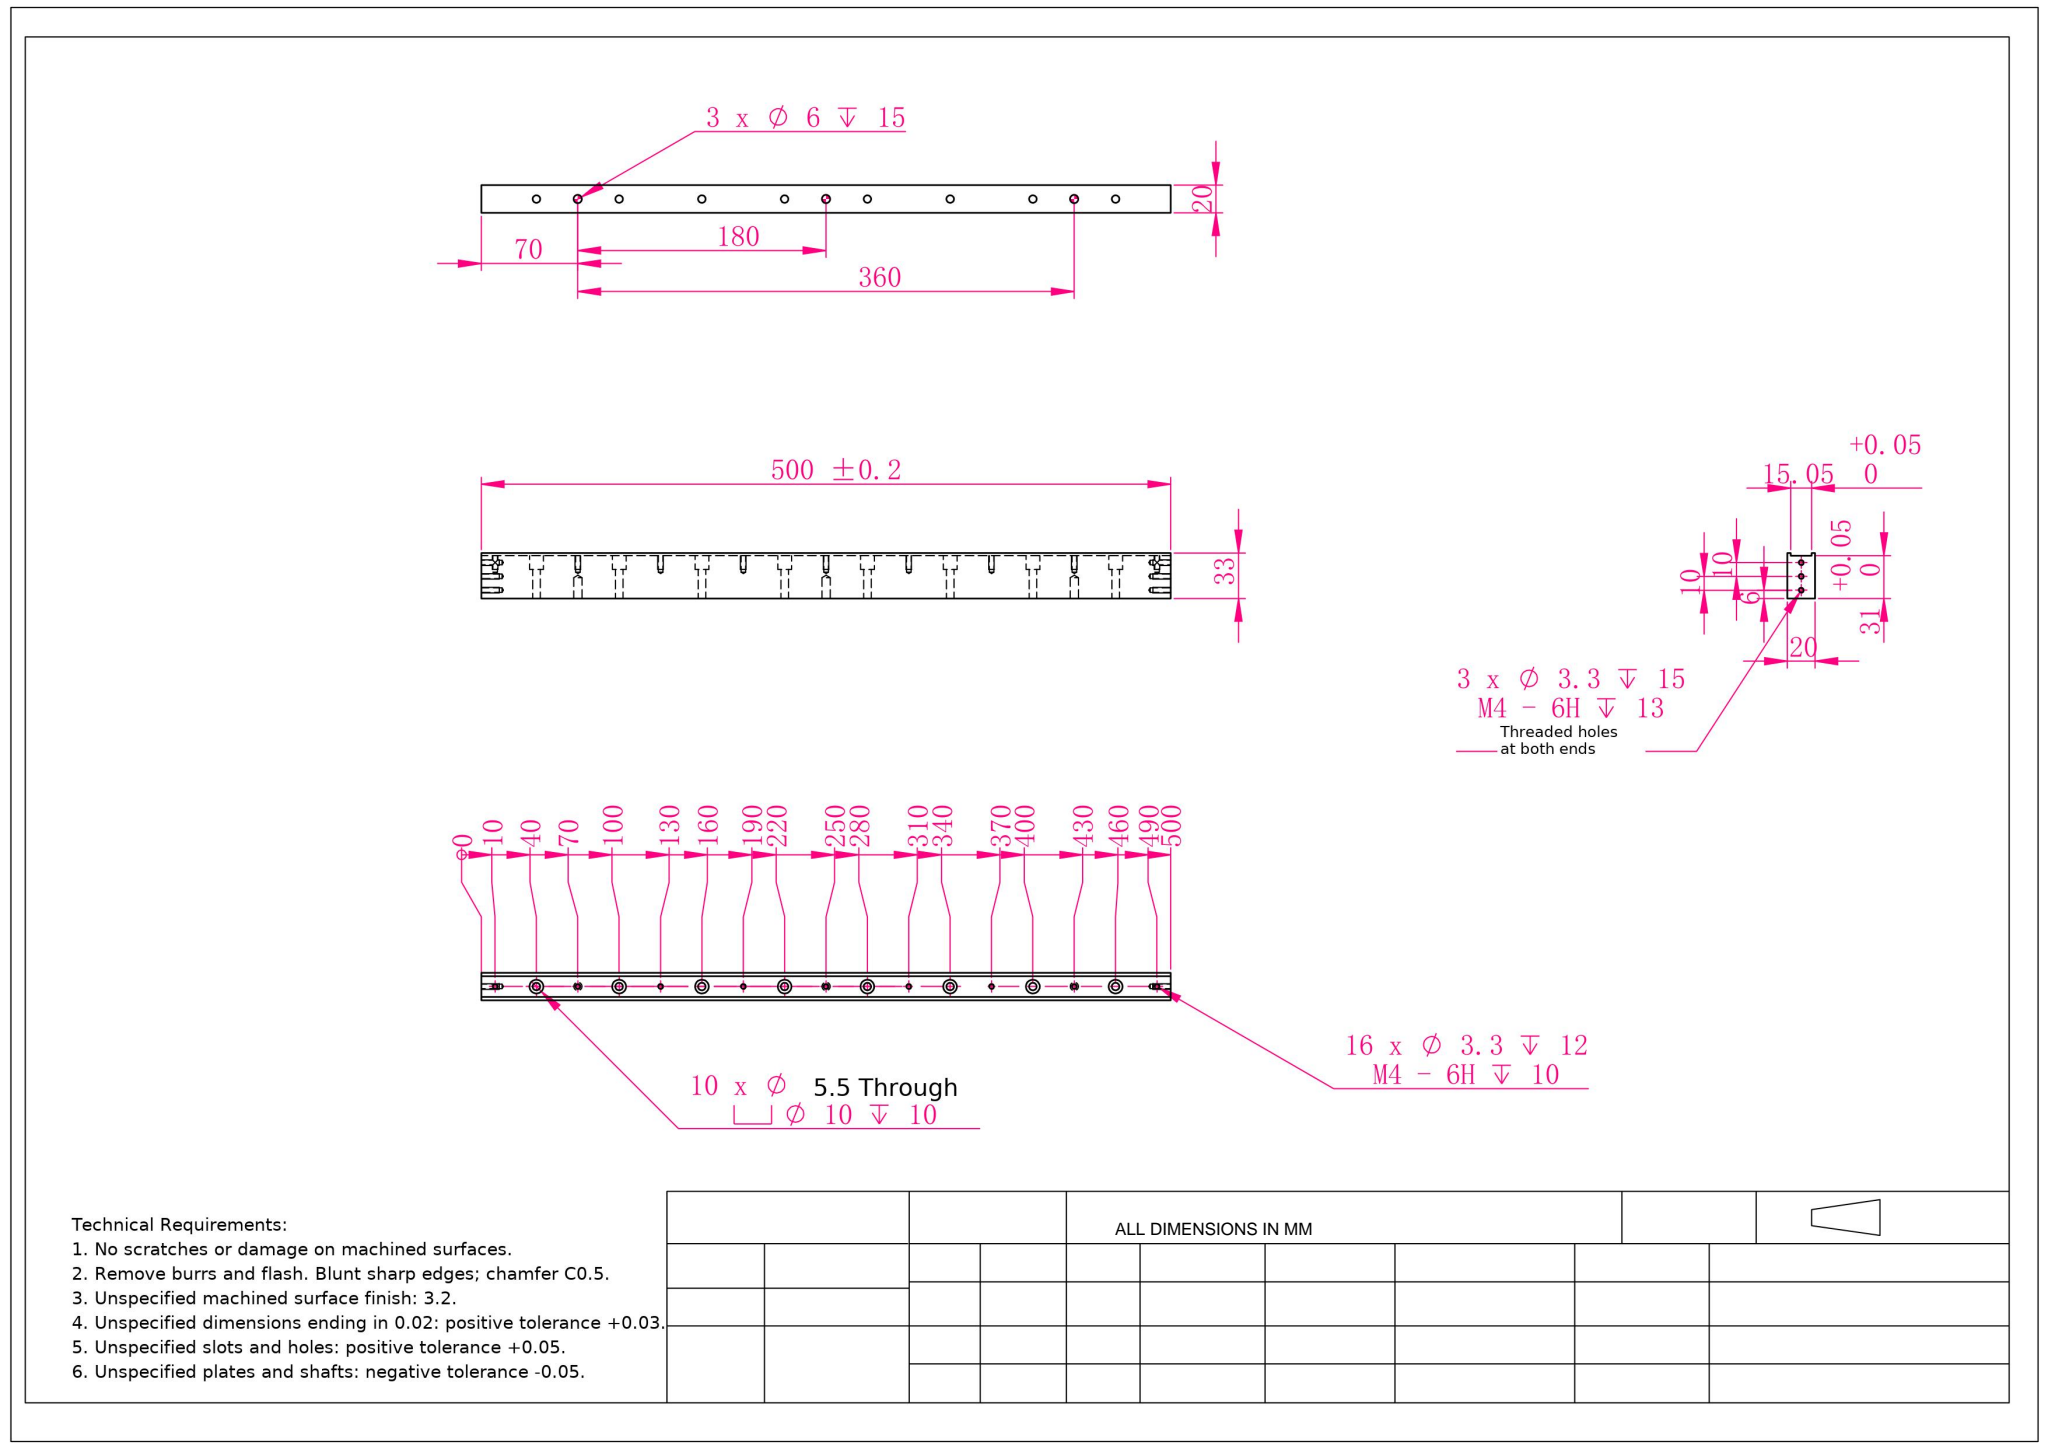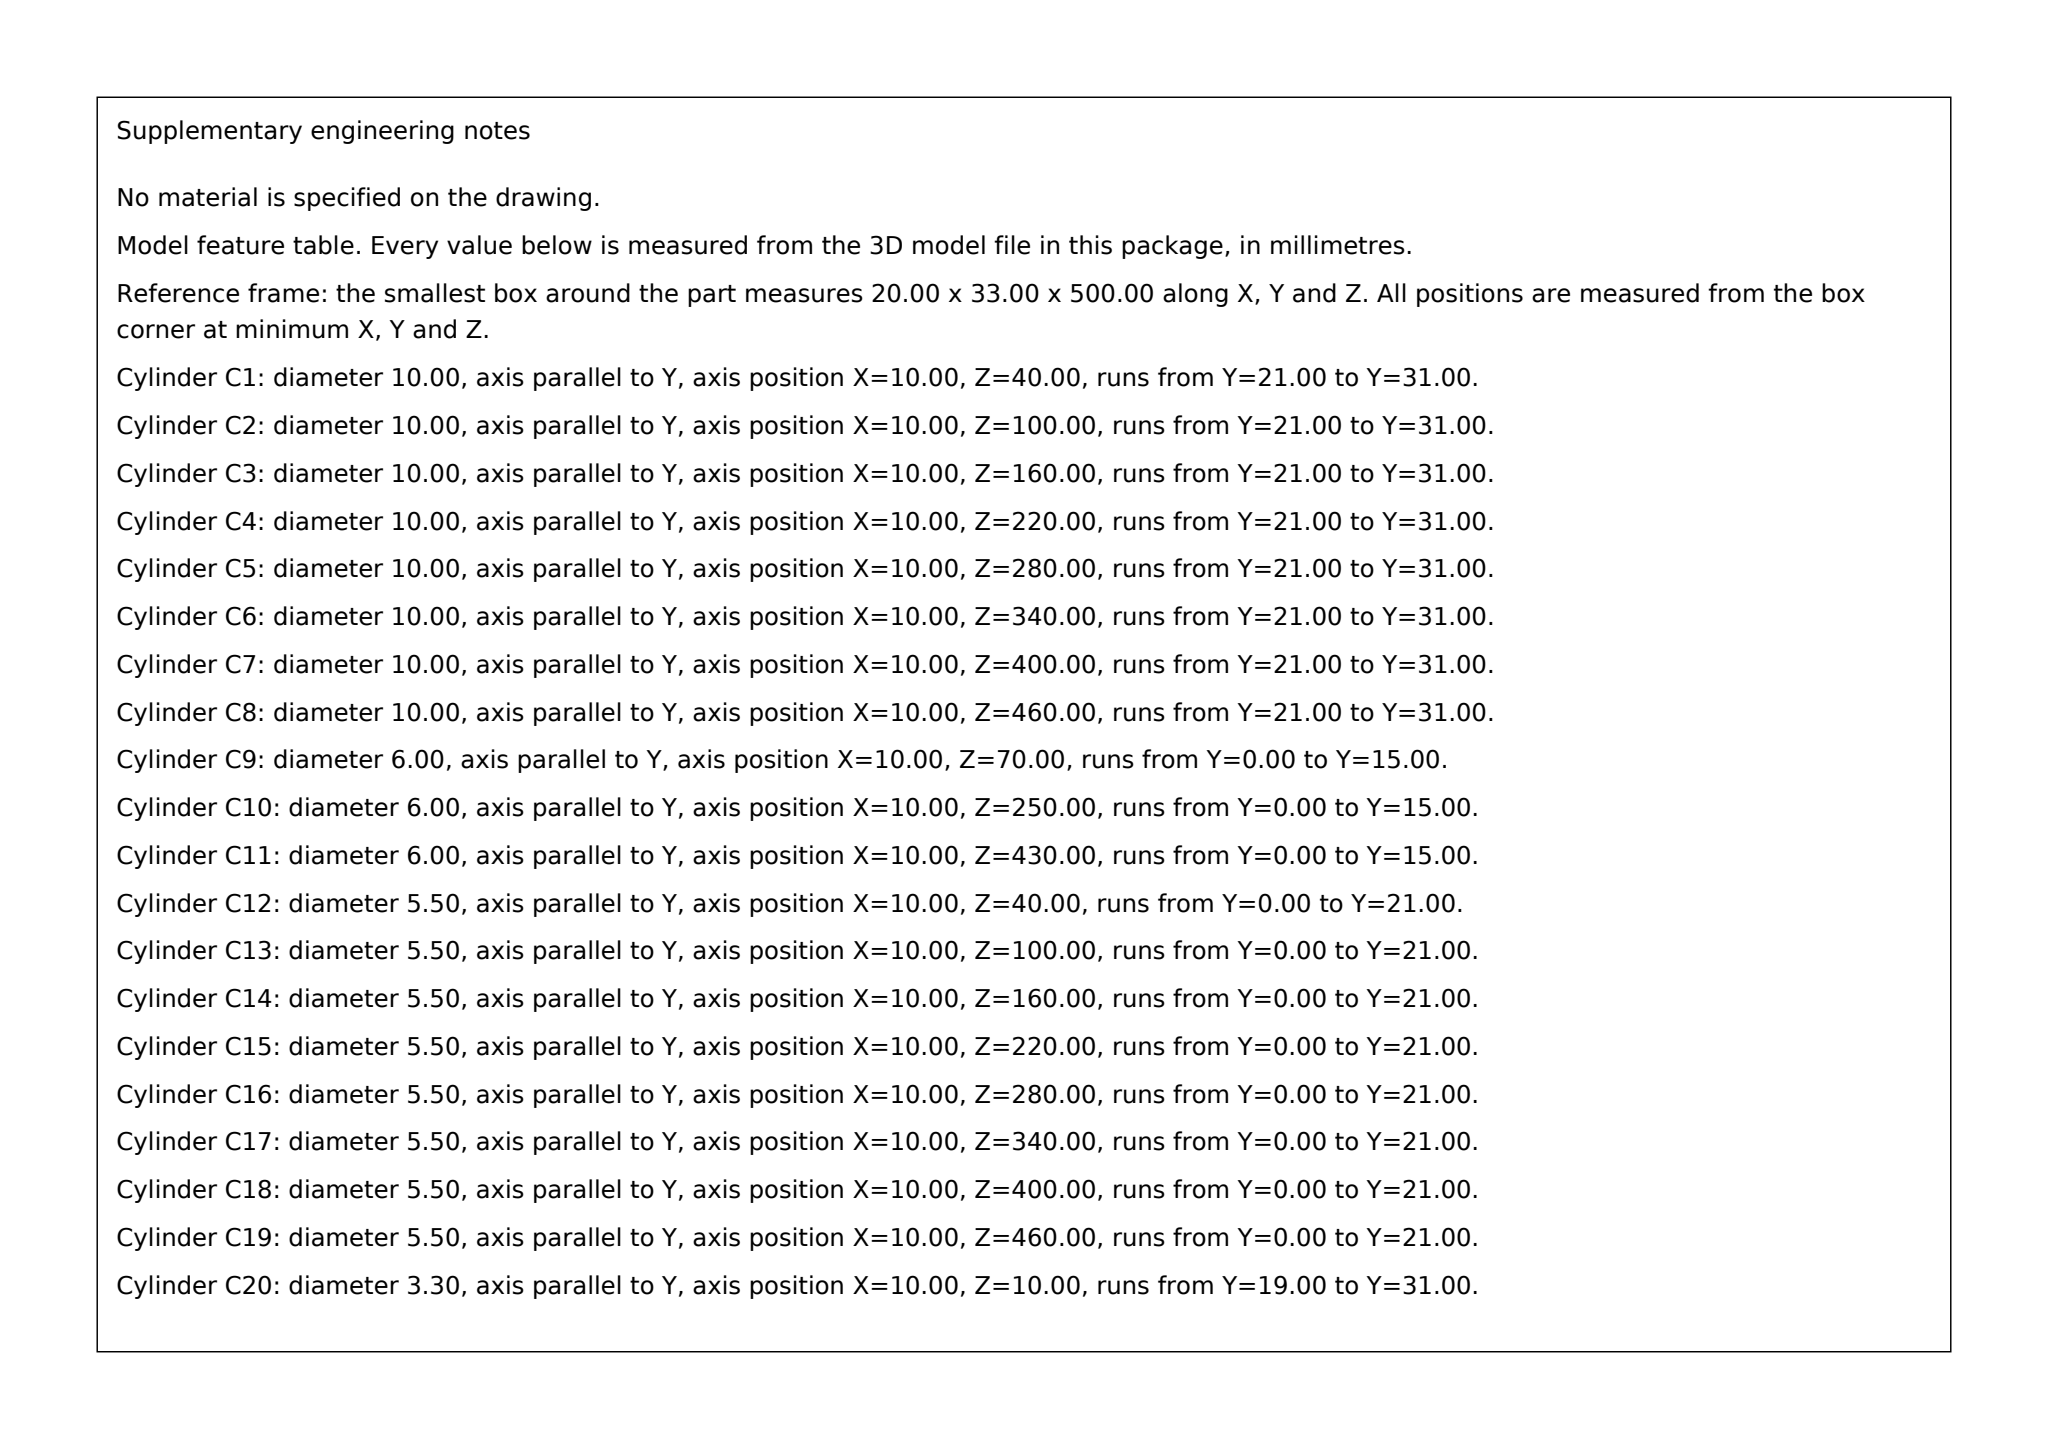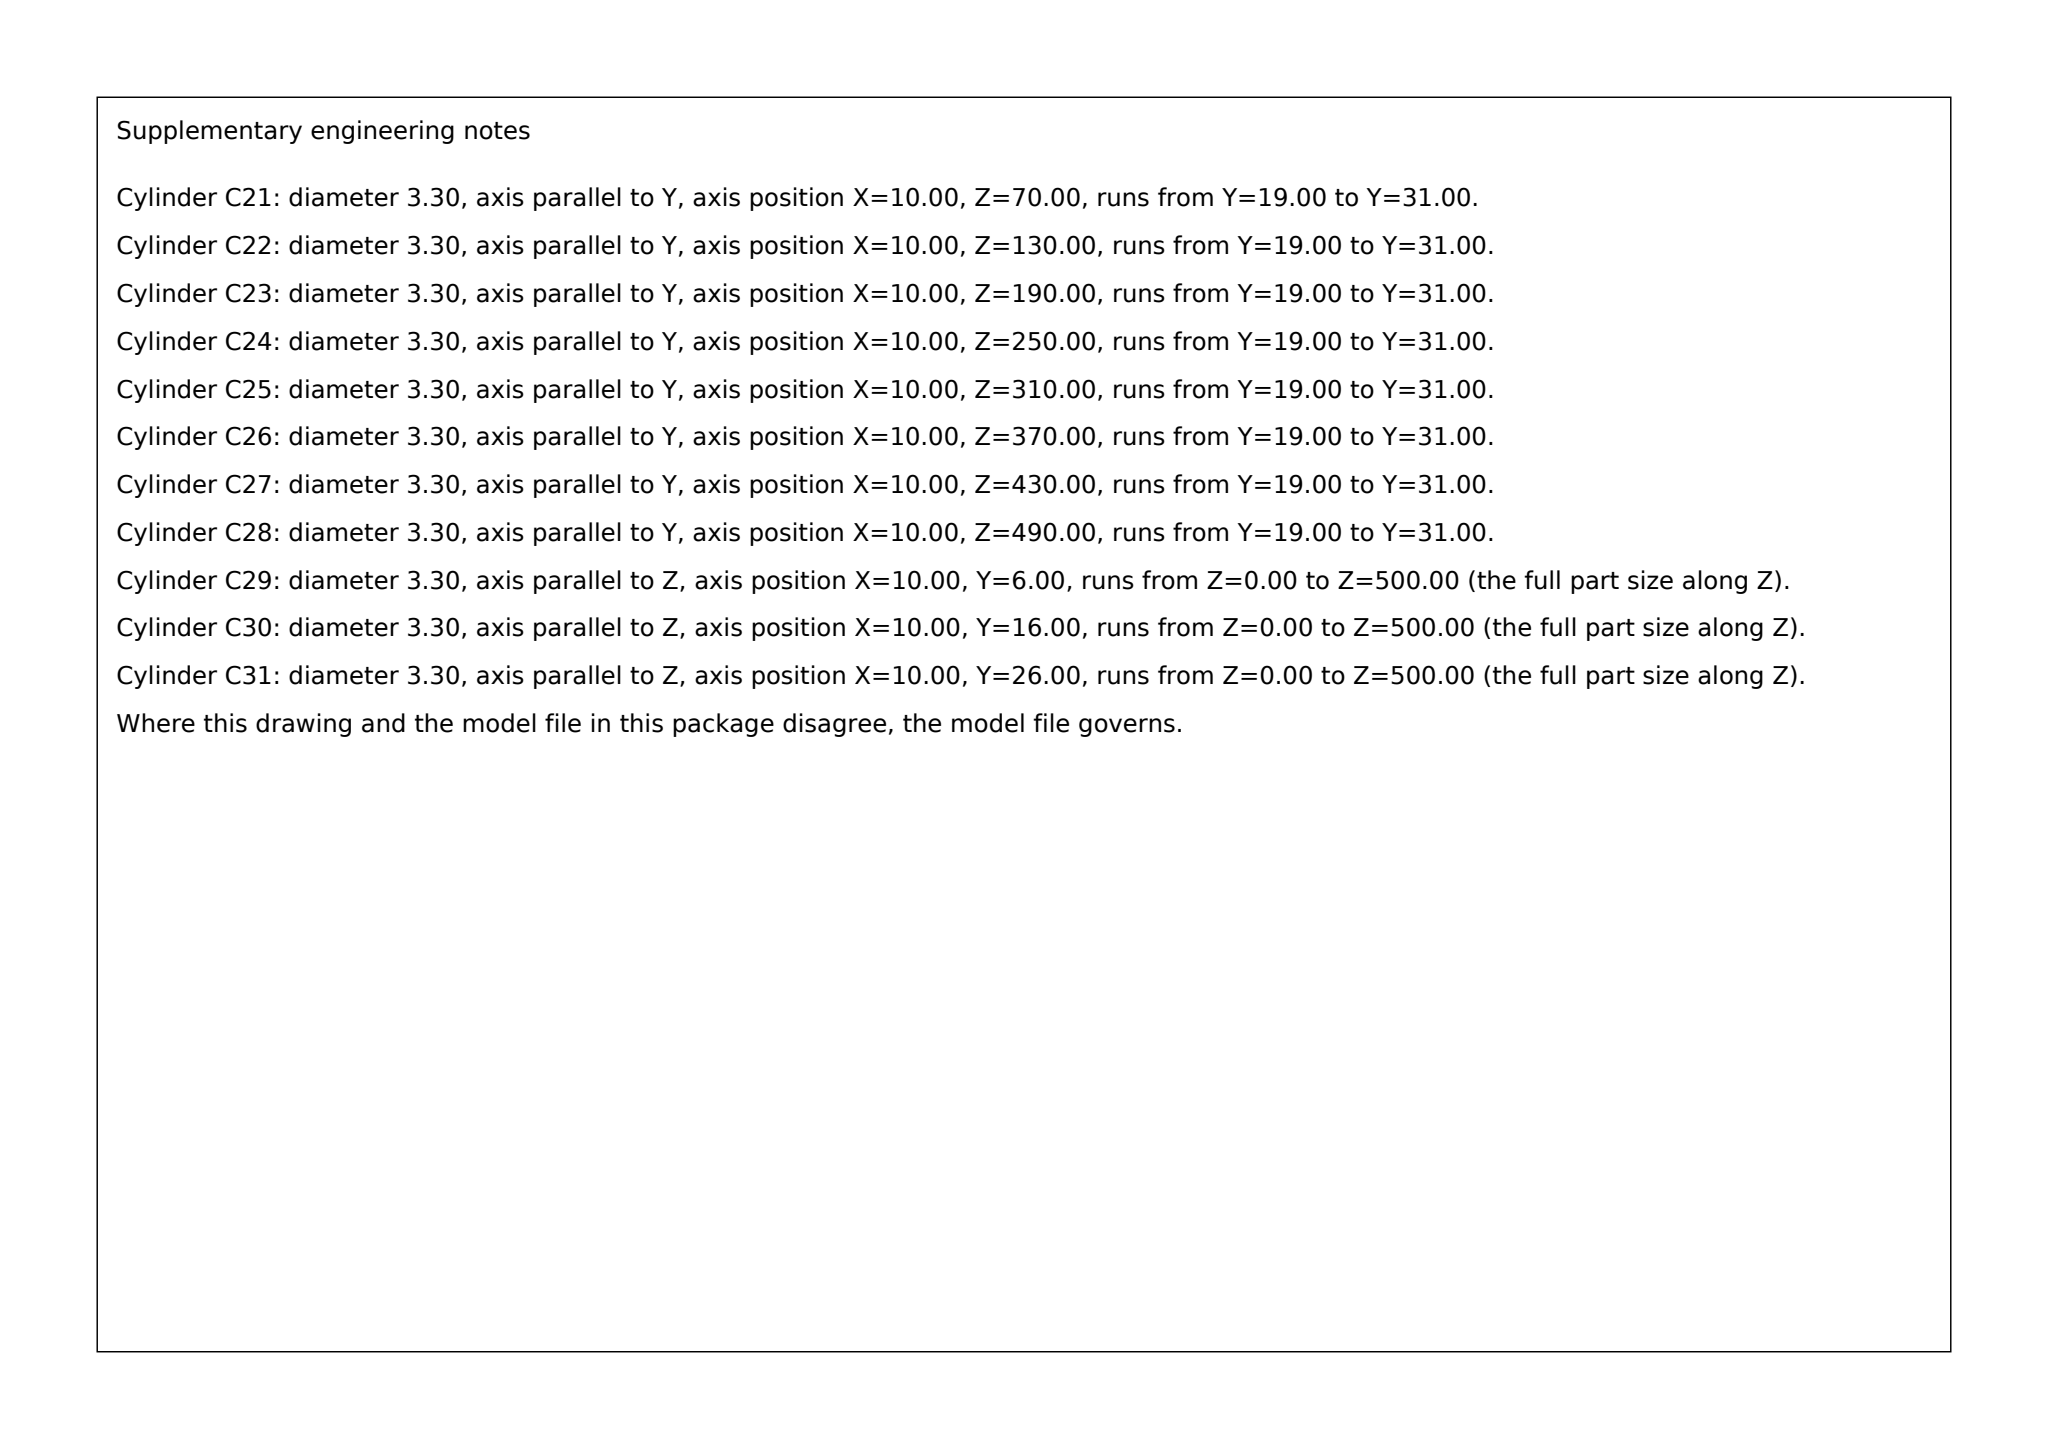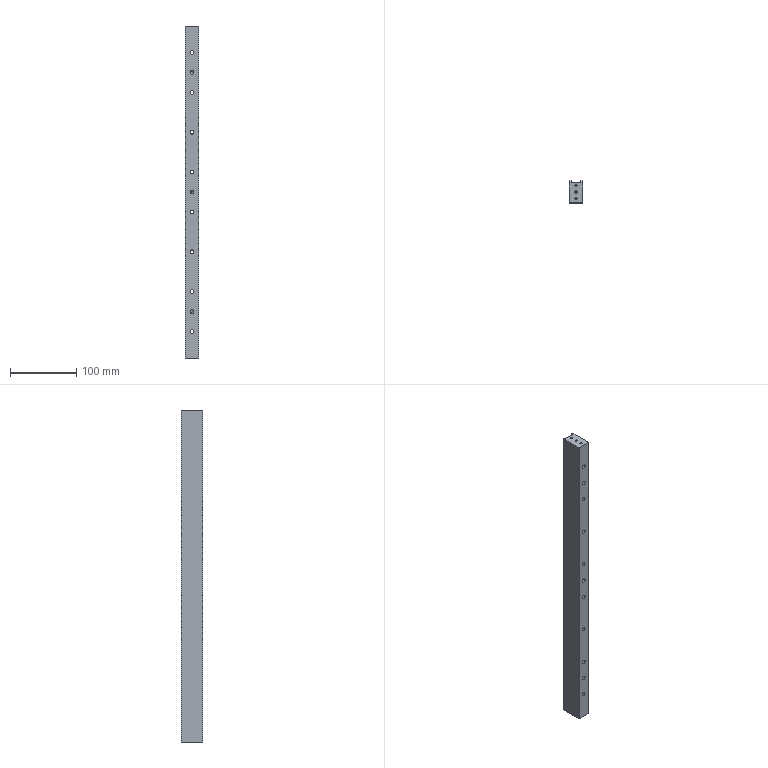Part | SolidWorks | mm | 1 solid | 130 faces | box 20 x 33 x 500 mm | volume 301664 mm3 | cylinder 76 | cone 36 | plane 18 | commonest cylinder face diameters 3.3 x38 10 x16 5.5 x16 6 x6
build123d program:
from build123d import *

# Parameters (mm, degrees)
BOSS_EXTRUDE1_DEPTH                             = 250
M4_TAPPED_HOLE2_D                               = 3.3
M4_TAPPED_HOLE2_DEPTH                           = 15
M4_TAPPED_HOLE2_TIP                             = 0.9914
M4_TAPPED_HOLE1_D                               = 3.3
M4_TAPPED_HOLE1_DEPTH                           = 15
M4_TAPPED_HOLE1_TIP                             = 0.9914
SIZE_MM_DOWEL_PIN_HOLE1_D                       = 6
SIZE_MM_DOWEL_PIN_HOLE1_DEPTH                   = 15
SIZE_MM_DOWEL_PIN_HOLE1_TIP                     = 1.803
M4_TAPPED_HOLE3_D                               = 3.3
M4_TAPPED_HOLE3_DEPTH                           = 12
M4_TAPPED_HOLE3_TIP                             = 0.9914
M5_HEX_SOCKET_HEAD_CAP_SCREW_CBORE1_D           = 5.5
M5_HEX_SOCKET_HEAD_CAP_SCREW_CBORE1_CBORE_D     = 10
M5_HEX_SOCKET_HEAD_CAP_SCREW_CBORE1_CBORE_DEPTH = 10


with BuildPart() as part:
    # Sketch1 → Boss-Extrude1 (new, symmetric)
    with BuildSketch(Plane.XY):
        Polygon((-10, -16.5), (10, -16.5), (10, 16.5), (7.525, 16.5), (7.525, 14.5), (-7.525, 14.5), (-7.525, 16.5), (-10, 16.5), align=None)
    extrude(amount=BOSS_EXTRUDE1_DEPTH, both=True)

    # M4 Tapped Hole2
    with Locations(Plane(origin=(0, 0, -250), x_dir=(1, 0, 0), z_dir=(0, 0, -1))):
        with Locations((0, -9.5), (0, 10.5), (0, 0.5)):
            Hole(M4_TAPPED_HOLE2_D / 2, depth=M4_TAPPED_HOLE2_DEPTH)
            with Locations((0, 0, -(M4_TAPPED_HOLE2_DEPTH + M4_TAPPED_HOLE2_TIP / 2))):  # 118° drill point
                Cone(0, M4_TAPPED_HOLE2_D / 2, M4_TAPPED_HOLE2_TIP, mode=Mode.SUBTRACT)

    # M4 Tapped Hole1
    with Locations(Plane.XY.offset(250)):
        with Locations((0, 9.5), (0, -10.5), (0, -0.5)):
            Hole(M4_TAPPED_HOLE1_D / 2, depth=M4_TAPPED_HOLE1_DEPTH)
            with Locations((0, 0, -(M4_TAPPED_HOLE1_DEPTH + M4_TAPPED_HOLE1_TIP / 2))):  # 118° drill point
                Cone(0, M4_TAPPED_HOLE1_D / 2, M4_TAPPED_HOLE1_TIP, mode=Mode.SUBTRACT)

    # Size mm Dowel Pin Hole1
    with Locations(Plane(origin=(0, -16.5, 0), x_dir=(-1, 0, 0), z_dir=(0, -1, 0))):
        with Locations((0, -180), (0, 180), (0, 0)):
            Hole(SIZE_MM_DOWEL_PIN_HOLE1_D / 2, depth=SIZE_MM_DOWEL_PIN_HOLE1_DEPTH)
            with Locations((0, 0, -(SIZE_MM_DOWEL_PIN_HOLE1_DEPTH + SIZE_MM_DOWEL_PIN_HOLE1_TIP / 2))):  # 118° drill point
                Cone(0, SIZE_MM_DOWEL_PIN_HOLE1_D / 2, SIZE_MM_DOWEL_PIN_HOLE1_TIP, mode=Mode.SUBTRACT)

    # M4 Tapped Hole3
    with Locations(Plane(origin=(0, 14.5, 0), x_dir=(1, 0, 0), z_dir=(0, 1, 0))):
        with Locations((0, -240), (0, -180), (0, -120), (0, -60), (0, 0), (0, 60), (0, 120), (0, 180), (0, 240), (0, 300), (0, 360), (0, 420), (0, 480), (0, 540), (0, 600), (0, 660)):
            Hole(M4_TAPPED_HOLE3_D / 2, depth=M4_TAPPED_HOLE3_DEPTH)
            with Locations((0, 0, -(M4_TAPPED_HOLE3_DEPTH + M4_TAPPED_HOLE3_TIP / 2))):  # 118° drill point
                Cone(0, M4_TAPPED_HOLE3_D / 2, M4_TAPPED_HOLE3_TIP, mode=Mode.SUBTRACT)

    # M5 Hex Socket Head Cap Screw CBORE1 (through all)
    with Locations(Plane(origin=(0, 14.5, 0), x_dir=(1, 0, 0), z_dir=(0, 1, 0))):
        with Locations((0, 210), (0, 150), (0, 30), (0, -30), (0, -90), (0, -210), (0, -150), (0, 90), (0, -270), (0, -330)):
            CounterBoreHole(M5_HEX_SOCKET_HEAD_CAP_SCREW_CBORE1_D / 2, M5_HEX_SOCKET_HEAD_CAP_SCREW_CBORE1_CBORE_D / 2, M5_HEX_SOCKET_HEAD_CAP_SCREW_CBORE1_CBORE_DEPTH)


solid = part.part